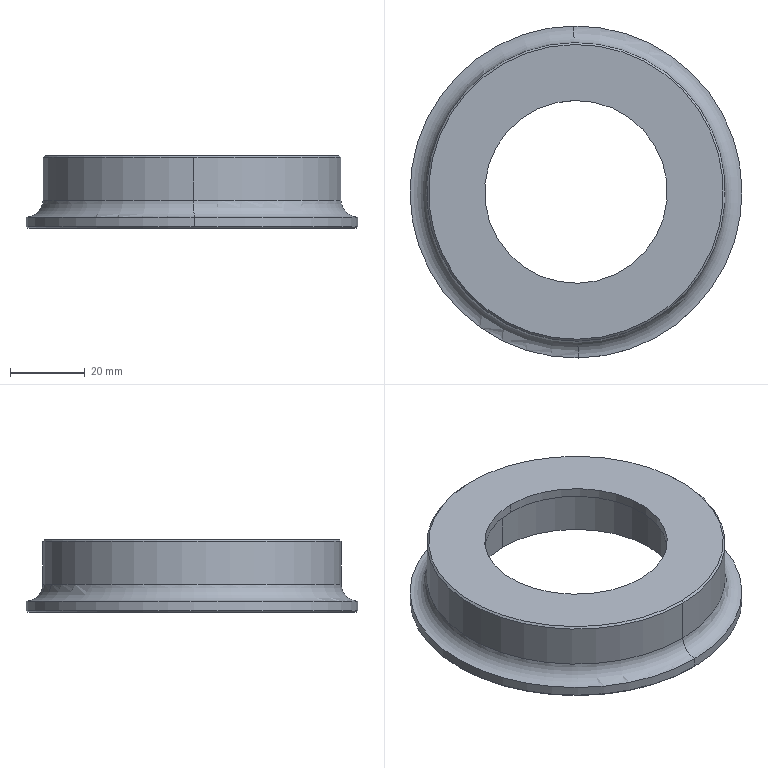Component | SolidWorks | 12AInnerSideWheel-EngravingAndMillingAxis-2_12AInnerSideWheel-2 | 1 solid | 20 faces | box 89 x 89 x 19.5 mm | volume 50313 mm3 | cylinder 10 | cone 4 | plane 4 | torus 2 | commonest cylinder face diameters 89 x2 73 x2 55 x2 49 x2 80 x2 | material Cr12MoV
build123d program:
from build123d import *

# Parameters (mm, degrees)
CHAMFER1_SIZE = 0.5
CHAMFER2_SIZE = 0.5


with BuildPart() as part:
    # Sketch1 → Revolve1 (revolve)
    with BuildSketch(Plane.XY, mode=Mode.PRIVATE) as revolve1_sk:
        with BuildLine():
            Line((27.5, 15.5), (27.5, 2.5))
            Line((27.5, 2.5), (24.5, 2.5))
            Line((24.5, 2.5), (24.5, 0))
            Line((24.5, 0), (40, 0))
            Line((40, 0), (40, 12))
            ThreePointArc((40, 12), (41.318, 15.182), (44.5, 16.5))
            Line((44.5, 16.5), (44.5, 19.5))
            Line((44.5, 19.5), (36.5, 19.5))
            Line((36.5, 19.5), (36.5, 15.5))
            Line((36.5, 15.5), (27.5, 15.5))
        make_face()
    revolve(revolve1_sk.sketch.rotate(Axis((0, 0, 0), (0, 1, 0)), 90), axis=Axis((0, 0, 0), (0, 1, 0)))

    # Chamfer1
    chamfer1_edges = [part.edges().sort_by_distance(p)[0] for p in [
        (0, 19.5, 44.5),
    ]]
    chamfer(chamfer1_edges, length=CHAMFER1_SIZE)

    # Chamfer2
    chamfer2_edges = [part.edges().sort_by_distance(p)[0] for p in [
        (0, 0, 40),
    ]]
    chamfer(chamfer2_edges, length=CHAMFER2_SIZE)


solid = part.part

# Placed as in the assembly
solid = solid.moved(Location((406.598, 137.038, 36.75), (-90, 0, 0)))
STEP:
#1=COLOUR_RGB('',0.7922,0.8196,0.9333);
#2=FILL_AREA_STYLE_COLOUR('',#1);
#3=FILL_AREA_STYLE('',(#2));
#4=SURFACE_STYLE_FILL_AREA(#3);
#5=SURFACE_SIDE_STYLE('',(#4));
#6=SURFACE_STYLE_USAGE(.BOTH.,#5);
#7=PRESENTATION_STYLE_ASSIGNMENT((#6));
#8=CARTESIAN_POINT('',(16.028,3.84,1.447));
#9=VERTEX_POINT('',#8);
#10=CARTESIAN_POINT('',(15.988,6.95,1.447));
#11=VERTEX_POINT('',#10);
#12=CARTESIAN_POINT('',(16.008,5.395,1.447));
#13=DIRECTION('',(-0.,-0.,1.));
#14=DIRECTION('',(0.01289,-0.9999,0.));
#15=AXIS2_PLACEMENT_3D('',#12,#13,#14);
#16=CIRCLE('',#15,1.555);
#17=EDGE_CURVE('',#9,#11,#16,.T.);
#18=ORIENTED_EDGE('',*,*,#17,.F.);
#19=CARTESIAN_POINT('',(16.028,3.821,1.427));
#20=VERTEX_POINT('',#19);
#21=CARTESIAN_POINT('',(16.028,3.84,1.447));
#22=DIRECTION('',(0.009113,-0.707,-0.7071));
#23=VECTOR('',#22,39.37);
#24=LINE('',#21,#23);
#25=EDGE_CURVE('',#9,#20,#24,.T.);
#26=ORIENTED_EDGE('',*,*,#25,.T.);
#27=CARTESIAN_POINT('',(15.988,6.97,1.427));
#28=VERTEX_POINT('',#27);
#29=CARTESIAN_POINT('',(16.008,5.395,1.427));
#30=DIRECTION('',(0.,0.,-1.));
#31=DIRECTION('',(0.01289,-0.9999,0.));
#32=AXIS2_PLACEMENT_3D('',#29,#30,#31);
#33=CIRCLE('',#32,1.575);
#34=EDGE_CURVE('',#28,#20,#33,.T.);
#35=ORIENTED_EDGE('',*,*,#34,.F.);
#36=CARTESIAN_POINT('',(15.988,6.95,1.447));
#37=DIRECTION('',(-0.009113,0.707,-0.7071));
#38=VECTOR('',#37,39.37);
#39=LINE('',#36,#38);
#40=EDGE_CURVE('',#11,#28,#39,.T.);
#41=ORIENTED_EDGE('',*,*,#40,.F.);
#42=EDGE_LOOP('',(#18,#26,#35,#41));
#43=FACE_OUTER_BOUND('',#42,.T.);
#44=CARTESIAN_POINT('',(16.008,5.395,1.447));
#45=DIRECTION('',(0.,0.,-1.));
#46=DIRECTION('',(-0.01289,0.9999,0.));
#47=AXIS2_PLACEMENT_3D('',#44,#45,#46);
#48=CONICAL_SURFACE('',#47,1.555,0.7854);
#49=ADVANCED_FACE('',(#43),#48,.T.);
#50=CARTESIAN_POINT('',(15.985,7.127,0.6791));
#51=VERTEX_POINT('',#50);
#52=CARTESIAN_POINT('',(16.03,3.663,0.6791));
#53=VERTEX_POINT('',#52);
#54=CARTESIAN_POINT('',(16.008,5.395,0.6791));
#55=DIRECTION('',(0.,0.,-1.));
#56=DIRECTION('',(-0.01289,0.9999,0.));
#57=AXIS2_PLACEMENT_3D('',#54,#55,#56);
#58=CIRCLE('',#57,1.732);
#59=EDGE_CURVE('',#51,#53,#58,.T.);
#60=ORIENTED_EDGE('',*,*,#59,.F.);
#61=CARTESIAN_POINT('',(15.985,7.147,0.6988));
#62=VERTEX_POINT('',#61);
#63=CARTESIAN_POINT('',(15.985,7.147,0.6988));
#64=DIRECTION('',(-0.009113,0.707,0.7071));
#65=VECTOR('',#64,39.37);
#66=LINE('',#63,#65);
#67=EDGE_CURVE('',#51,#62,#66,.T.);
#68=ORIENTED_EDGE('',*,*,#67,.T.);
#69=CARTESIAN_POINT('',(16.03,3.643,0.6988));
#70=VERTEX_POINT('',#69);
#71=CARTESIAN_POINT('',(16.008,5.395,0.6988));
#72=DIRECTION('',(-0.,-0.,1.));
#73=DIRECTION('',(-0.01289,0.9999,0.));
#74=AXIS2_PLACEMENT_3D('',#71,#72,#73);
#75=CIRCLE('',#74,1.752);
#76=EDGE_CURVE('',#70,#62,#75,.T.);
#77=ORIENTED_EDGE('',*,*,#76,.F.);
#78=CARTESIAN_POINT('',(16.03,3.643,0.6988));
#79=DIRECTION('',(0.009113,-0.707,0.7071));
#80=VECTOR('',#79,39.37);
#81=LINE('',#78,#80);
#82=EDGE_CURVE('',#53,#70,#81,.T.);
#83=ORIENTED_EDGE('',*,*,#82,.F.);
#84=EDGE_LOOP('',(#60,#68,#77,#83));
#85=FACE_OUTER_BOUND('',#84,.T.);
#86=CARTESIAN_POINT('',(16.008,5.395,0.6988));
#87=DIRECTION('',(-0.,-0.,1.));
#88=DIRECTION('',(0.01289,-0.9999,0.));
#89=AXIS2_PLACEMENT_3D('',#86,#87,#88);
#90=CONICAL_SURFACE('',#89,1.752,0.7854);
#91=ADVANCED_FACE('',(#85),#90,.T.);
#92=ORIENTED_EDGE('',*,*,#76,.T.);
#93=CARTESIAN_POINT('',(15.985,7.147,0.7972));
#94=VERTEX_POINT('',#93);
#95=CARTESIAN_POINT('',(15.985,7.147,1.447));
#96=DIRECTION('',(-0.,-0.,1.));
#97=VECTOR('',#96,39.37);
#98=LINE('',#95,#97);
#99=EDGE_CURVE('',#62,#94,#98,.T.);
#100=ORIENTED_EDGE('',*,*,#99,.T.);
#101=CARTESIAN_POINT('',(16.03,3.643,0.7972));
#102=VERTEX_POINT('',#101);
#103=CARTESIAN_POINT('',(16.008,5.395,0.7972));
#104=DIRECTION('',(-0.,-0.,1.));
#105=DIRECTION('',(0.01289,-0.9999,0.));
#106=AXIS2_PLACEMENT_3D('',#103,#104,#105);
#107=CIRCLE('',#106,1.752);
#108=EDGE_CURVE('',#102,#94,#107,.T.);
#109=ORIENTED_EDGE('',*,*,#108,.F.);
#110=CARTESIAN_POINT('',(16.03,3.643,1.447));
#111=DIRECTION('',(-0.,-0.,1.));
#112=VECTOR('',#111,39.37);
#113=LINE('',#110,#112);
#114=EDGE_CURVE('',#70,#102,#113,.T.);
#115=ORIENTED_EDGE('',*,*,#114,.F.);
#116=EDGE_LOOP('',(#92,#100,#109,#115));
#117=FACE_OUTER_BOUND('',#116,.T.);
#118=CARTESIAN_POINT('',(16.008,5.395,1.447));
#119=DIRECTION('',(-0.,-0.,1.));
#120=DIRECTION('',(0.01289,-0.9999,0.));
#121=AXIS2_PLACEMENT_3D('',#118,#119,#120);
#122=CYLINDRICAL_SURFACE('',#121,1.752);
#123=ADVANCED_FACE('',(#117),#122,.T.);
#124=CARTESIAN_POINT('',(15.989,6.832,0.6791));
#125=VERTEX_POINT('',#124);
#126=CARTESIAN_POINT('',(16.026,3.958,0.6791));
#127=VERTEX_POINT('',#126);
#128=CARTESIAN_POINT('',(16.008,5.395,0.6791));
#129=DIRECTION('',(-0.,-0.,1.));
#130=DIRECTION('',(0.01289,-0.9999,0.));
#131=AXIS2_PLACEMENT_3D('',#128,#129,#130);
#132=CIRCLE('',#131,1.437);
#133=EDGE_CURVE('',#125,#127,#132,.T.);
#134=ORIENTED_EDGE('',*,*,#133,.F.);
#135=CARTESIAN_POINT('',(15.989,6.832,0.8366));
#136=VERTEX_POINT('',#135);
#137=CARTESIAN_POINT('',(15.989,6.832,1.447));
#138=DIRECTION('',(-0.,-0.,1.));
#139=VECTOR('',#138,39.37);
#140=LINE('',#137,#139);
#141=EDGE_CURVE('',#125,#136,#140,.T.);
#142=ORIENTED_EDGE('',*,*,#141,.T.);
#143=CARTESIAN_POINT('',(16.026,3.958,0.8366));
#144=VERTEX_POINT('',#143);
#145=CARTESIAN_POINT('',(16.008,5.395,0.8366));
#146=DIRECTION('',(-0.,-0.,1.));
#147=DIRECTION('',(0.01289,-0.9999,0.));
#148=AXIS2_PLACEMENT_3D('',#145,#146,#147);
#149=CIRCLE('',#148,1.437);
#150=EDGE_CURVE('',#136,#144,#149,.T.);
#151=ORIENTED_EDGE('',*,*,#150,.T.);
#152=CARTESIAN_POINT('',(16.026,3.958,1.447));
#153=DIRECTION('',(-0.,-0.,1.));
#154=VECTOR('',#153,39.37);
#155=LINE('',#152,#154);
#156=EDGE_CURVE('',#127,#144,#155,.T.);
#157=ORIENTED_EDGE('',*,*,#156,.F.);
#158=EDGE_LOOP('',(#134,#142,#151,#157));
#159=FACE_OUTER_BOUND('',#158,.T.);
#160=CARTESIAN_POINT('',(16.008,5.395,1.447));
#161=DIRECTION('',(-0.,-0.,1.));
#162=DIRECTION('',(0.01289,-0.9999,0.));
#163=AXIS2_PLACEMENT_3D('',#160,#161,#162);
#164=CYLINDRICAL_SURFACE('',#163,1.437);
#165=ADVANCED_FACE('',(#159),#164,.F.);
#166=CARTESIAN_POINT('',(15.994,6.478,0.8366));
#167=VERTEX_POINT('',#166);
#168=CARTESIAN_POINT('',(16.022,4.313,0.8366));
#169=VERTEX_POINT('',#168);
#170=CARTESIAN_POINT('',(16.008,5.395,0.8366));
#171=DIRECTION('',(-0.,-0.,1.));
#172=DIRECTION('',(0.01289,-0.9999,0.));
#173=AXIS2_PLACEMENT_3D('',#170,#171,#172);
#174=CIRCLE('',#173,1.083);
#175=EDGE_CURVE('',#167,#169,#174,.T.);
#176=ORIENTED_EDGE('',*,*,#175,.F.);
#177=CARTESIAN_POINT('',(15.994,6.478,1.348));
#178=VERTEX_POINT('',#177);
#179=CARTESIAN_POINT('',(15.994,6.478,1.447));
#180=DIRECTION('',(-0.,-0.,1.));
#181=VECTOR('',#180,39.37);
#182=LINE('',#179,#181);
#183=EDGE_CURVE('',#167,#178,#182,.T.);
#184=ORIENTED_EDGE('',*,*,#183,.T.);
#185=CARTESIAN_POINT('',(16.022,4.313,1.348));
#186=VERTEX_POINT('',#185);
#187=CARTESIAN_POINT('',(16.008,5.395,1.348));
#188=DIRECTION('',(-0.,-0.,1.));
#189=DIRECTION('',(0.01289,-0.9999,0.));
#190=AXIS2_PLACEMENT_3D('',#187,#188,#189);
#191=CIRCLE('',#190,1.083);
#192=EDGE_CURVE('',#178,#186,#191,.T.);
#193=ORIENTED_EDGE('',*,*,#192,.T.);
#194=CARTESIAN_POINT('',(16.022,4.313,1.447));
#195=DIRECTION('',(-0.,-0.,1.));
#196=VECTOR('',#195,39.37);
#197=LINE('',#194,#196);
#198=EDGE_CURVE('',#169,#186,#197,.T.);
#199=ORIENTED_EDGE('',*,*,#198,.F.);
#200=EDGE_LOOP('',(#176,#184,#193,#199));
#201=FACE_OUTER_BOUND('',#200,.T.);
#202=CARTESIAN_POINT('',(16.008,5.395,1.447));
#203=DIRECTION('',(-0.,-0.,1.));
#204=DIRECTION('',(0.01289,-0.9999,0.));
#205=AXIS2_PLACEMENT_3D('',#202,#203,#204);
#206=CYLINDRICAL_SURFACE('',#205,1.083);
#207=ADVANCED_FACE('',(#201),#206,.F.);
#208=CARTESIAN_POINT('',(15.995,6.36,1.348));
#209=VERTEX_POINT('',#208);
#210=CARTESIAN_POINT('',(16.02,4.431,1.348));
#211=VERTEX_POINT('',#210);
#212=CARTESIAN_POINT('',(16.008,5.395,1.348));
#213=DIRECTION('',(-0.,-0.,1.));
#214=DIRECTION('',(0.01289,-0.9999,0.));
#215=AXIS2_PLACEMENT_3D('',#212,#213,#214);
#216=CIRCLE('',#215,0.9646);
#217=EDGE_CURVE('',#209,#211,#216,.T.);
#218=ORIENTED_EDGE('',*,*,#217,.F.);
#219=CARTESIAN_POINT('',(15.995,6.36,1.447));
#220=VERTEX_POINT('',#219);
#221=CARTESIAN_POINT('',(15.995,6.36,1.447));
#222=DIRECTION('',(-0.,-0.,1.));
#223=VECTOR('',#222,39.37);
#224=LINE('',#221,#223);
#225=EDGE_CURVE('',#209,#220,#224,.T.);
#226=ORIENTED_EDGE('',*,*,#225,.T.);
#227=CARTESIAN_POINT('',(16.02,4.431,1.447));
#228=VERTEX_POINT('',#227);
#229=CARTESIAN_POINT('',(16.008,5.395,1.447));
#230=DIRECTION('',(-0.,-0.,1.));
#231=DIRECTION('',(0.01289,-0.9999,0.));
#232=AXIS2_PLACEMENT_3D('',#229,#230,#231);
#233=CIRCLE('',#232,0.9646);
#234=EDGE_CURVE('',#220,#228,#233,.T.);
#235=ORIENTED_EDGE('',*,*,#234,.T.);
#236=CARTESIAN_POINT('',(16.02,4.431,1.447));
#237=DIRECTION('',(-0.,-0.,1.));
#238=VECTOR('',#237,39.37);
#239=LINE('',#236,#238);
#240=EDGE_CURVE('',#211,#228,#239,.T.);
#241=ORIENTED_EDGE('',*,*,#240,.F.);
#242=EDGE_LOOP('',(#218,#226,#235,#241));
#243=FACE_OUTER_BOUND('',#242,.T.);
#244=CARTESIAN_POINT('',(16.008,5.395,1.447));
#245=DIRECTION('',(-0.,-0.,1.));
#246=DIRECTION('',(0.01289,-0.9999,0.));
#247=AXIS2_PLACEMENT_3D('',#244,#245,#246);
#248=CYLINDRICAL_SURFACE('',#247,0.9646);
#249=ADVANCED_FACE('',(#243),#248,.F.);
#250=CARTESIAN_POINT('',(16.028,3.821,0.9744));
#251=VERTEX_POINT('',#250);
#252=CARTESIAN_POINT('',(15.988,6.97,0.9744));
#253=VERTEX_POINT('',#252);
#254=CARTESIAN_POINT('',(16.008,5.395,0.9744));
#255=DIRECTION('',(-0.,-0.,1.));
#256=DIRECTION('',(0.01289,-0.9999,0.));
#257=AXIS2_PLACEMENT_3D('',#254,#255,#256);
#258=CIRCLE('',#257,1.575);
#259=EDGE_CURVE('',#251,#253,#258,.T.);
#260=ORIENTED_EDGE('',*,*,#259,.T.);
#261=CARTESIAN_POINT('',(15.988,6.97,1.447));
#262=DIRECTION('',(-0.,-0.,1.));
#263=VECTOR('',#262,39.37);
#264=LINE('',#261,#263);
#265=EDGE_CURVE('',#253,#28,#264,.T.);
#266=ORIENTED_EDGE('',*,*,#265,.T.);
#267=ORIENTED_EDGE('',*,*,#34,.T.);
#268=CARTESIAN_POINT('',(16.028,3.821,1.447));
#269=DIRECTION('',(-0.,-0.,1.));
#270=VECTOR('',#269,39.37);
#271=LINE('',#268,#270);
#272=EDGE_CURVE('',#251,#20,#271,.T.);
#273=ORIENTED_EDGE('',*,*,#272,.F.);
#274=EDGE_LOOP('',(#260,#266,#267,#273));
#275=FACE_OUTER_BOUND('',#274,.T.);
#276=CARTESIAN_POINT('',(16.008,5.395,1.447));
#277=DIRECTION('',(-0.,-0.,1.));
#278=DIRECTION('',(0.01289,-0.9999,0.));
#279=AXIS2_PLACEMENT_3D('',#276,#277,#278);
#280=CYLINDRICAL_SURFACE('',#279,1.575);
#281=ADVANCED_FACE('',(#275),#280,.T.);
#282=CARTESIAN_POINT('',(16.008,5.395,0.9744));
#283=DIRECTION('',(-0.,-0.,1.));
#284=DIRECTION('',(0.01289,-0.9999,0.));
#285=AXIS2_PLACEMENT_3D('',#282,#283,#284);
#286=CIRCLE('',#285,1.575);
#287=EDGE_CURVE('',#253,#251,#286,.T.);
#288=ORIENTED_EDGE('',*,*,#287,.F.);
#289=CARTESIAN_POINT('',(15.985,7.147,0.9744));
#290=DIRECTION('',(0.9999,0.01289,0.));
#291=DIRECTION('',(-0.01289,0.9999,0.));
#292=AXIS2_PLACEMENT_3D('',#289,#290,#291);
#293=CIRCLE('',#292,0.1772);
#294=EDGE_CURVE('',#253,#94,#293,.T.);
#295=ORIENTED_EDGE('',*,*,#294,.T.);
#296=CARTESIAN_POINT('',(16.008,5.395,0.7972));
#297=DIRECTION('',(-0.,-0.,1.));
#298=DIRECTION('',(0.01289,-0.9999,0.));
#299=AXIS2_PLACEMENT_3D('',#296,#297,#298);
#300=CIRCLE('',#299,1.752);
#301=EDGE_CURVE('',#94,#102,#300,.T.);
#302=ORIENTED_EDGE('',*,*,#301,.T.);
#303=CARTESIAN_POINT('',(16.03,3.643,0.9744));
#304=DIRECTION('',(-0.9999,-0.01289,-0.));
#305=DIRECTION('',(0.01289,-0.9999,0.));
#306=AXIS2_PLACEMENT_3D('',#303,#304,#305);
#307=CIRCLE('',#306,0.1772);
#308=EDGE_CURVE('',#251,#102,#307,.T.);
#309=ORIENTED_EDGE('',*,*,#308,.F.);
#310=EDGE_LOOP('',(#288,#295,#302,#309));
#311=FACE_OUTER_BOUND('',#310,.T.);
#312=CARTESIAN_POINT('',(16.008,5.395,0.9744));
#313=DIRECTION('',(-0.,-0.,1.));
#314=DIRECTION('',(0.01289,-0.9999,-0.));
#315=AXIS2_PLACEMENT_3D('',#312,#313,#314);
#316=TOROIDAL_SURFACE('',#315,1.752,0.1772);
#317=ADVANCED_FACE('',(#311),#316,.F.);
#318=ORIENTED_EDGE('',*,*,#294,.F.);
#319=ORIENTED_EDGE('',*,*,#259,.F.);
#320=ORIENTED_EDGE('',*,*,#308,.T.);
#321=ORIENTED_EDGE('',*,*,#108,.T.);
#322=EDGE_LOOP('',(#318,#319,#320,#321));
#323=FACE_OUTER_BOUND('',#322,.T.);
#324=CARTESIAN_POINT('',(16.008,5.395,0.9744));
#325=DIRECTION('',(-0.,-0.,1.));
#326=DIRECTION('',(0.01289,-0.9999,-0.));
#327=AXIS2_PLACEMENT_3D('',#324,#325,#326);
#328=TOROIDAL_SURFACE('',#327,1.752,0.1772);
#329=ADVANCED_FACE('',(#323),#328,.F.);
#330=ORIENTED_EDGE('',*,*,#265,.F.);
#331=ORIENTED_EDGE('',*,*,#287,.T.);
#332=ORIENTED_EDGE('',*,*,#272,.T.);
#333=CARTESIAN_POINT('',(16.008,5.395,1.427));
#334=DIRECTION('',(0.,0.,-1.));
#335=DIRECTION('',(0.01289,-0.9999,0.));
#336=AXIS2_PLACEMENT_3D('',#333,#334,#335);
#337=CIRCLE('',#336,1.575);
#338=EDGE_CURVE('',#20,#28,#337,.T.);
#339=ORIENTED_EDGE('',*,*,#338,.T.);
#340=EDGE_LOOP('',(#330,#331,#332,#339));
#341=FACE_OUTER_BOUND('',#340,.T.);
#342=CARTESIAN_POINT('',(16.008,5.395,1.447));
#343=DIRECTION('',(-0.,-0.,1.));
#344=DIRECTION('',(0.01289,-0.9999,0.));
#345=AXIS2_PLACEMENT_3D('',#342,#343,#344);
#346=CYLINDRICAL_SURFACE('',#345,1.575);
#347=ADVANCED_FACE('',(#341),#346,.T.);
#348=CARTESIAN_POINT('',(16.008,5.395,1.447));
#349=DIRECTION('',(-0.,-0.,1.));
#350=DIRECTION('',(0.01289,-0.9999,0.));
#351=AXIS2_PLACEMENT_3D('',#348,#349,#350);
#352=CIRCLE('',#351,1.555);
#353=EDGE_CURVE('',#11,#9,#352,.T.);
#354=ORIENTED_EDGE('',*,*,#353,.T.);
#355=ORIENTED_EDGE('',*,*,#17,.T.);
#356=EDGE_LOOP('',(#354,#355));
#357=FACE_OUTER_BOUND('',#356,.T.);
#358=CARTESIAN_POINT('',(16.008,5.395,1.447));
#359=DIRECTION('',(-0.,-0.,1.));
#360=DIRECTION('',(0.01289,-0.9999,0.));
#361=AXIS2_PLACEMENT_3D('',#358,#359,#360);
#362=CIRCLE('',#361,0.9646);
#363=EDGE_CURVE('',#228,#220,#362,.T.);
#364=ORIENTED_EDGE('',*,*,#363,.F.);
#365=ORIENTED_EDGE('',*,*,#234,.F.);
#366=EDGE_LOOP('',(#364,#365));
#367=FACE_BOUND('',#366,.T.);
#368=CARTESIAN_POINT('',(16.972,5.408,1.447));
#369=DIRECTION('',(-0.,-0.,1.));
#370=DIRECTION('',(0.01289,-0.9999,-0.));
#371=AXIS2_PLACEMENT_3D('',#368,#369,#370);
#372=PLANE('',#371);
#373=ADVANCED_FACE('',(#357,#367),#372,.T.);
#374=ORIENTED_EDGE('',*,*,#225,.F.);
#375=CARTESIAN_POINT('',(16.008,5.395,1.348));
#376=DIRECTION('',(-0.,-0.,1.));
#377=DIRECTION('',(0.01289,-0.9999,0.));
#378=AXIS2_PLACEMENT_3D('',#375,#376,#377);
#379=CIRCLE('',#378,0.9646);
#380=EDGE_CURVE('',#211,#209,#379,.T.);
#381=ORIENTED_EDGE('',*,*,#380,.F.);
#382=ORIENTED_EDGE('',*,*,#240,.T.);
#383=ORIENTED_EDGE('',*,*,#363,.T.);
#384=EDGE_LOOP('',(#374,#381,#382,#383));
#385=FACE_OUTER_BOUND('',#384,.T.);
#386=CARTESIAN_POINT('',(16.008,5.395,1.447));
#387=DIRECTION('',(-0.,-0.,1.));
#388=DIRECTION('',(0.01289,-0.9999,0.));
#389=AXIS2_PLACEMENT_3D('',#386,#387,#388);
#390=CYLINDRICAL_SURFACE('',#389,0.9646);
#391=ADVANCED_FACE('',(#385),#390,.F.);
#392=ORIENTED_EDGE('',*,*,#380,.T.);
#393=ORIENTED_EDGE('',*,*,#217,.T.);
#394=EDGE_LOOP('',(#392,#393));
#395=FACE_BOUND('',#394,.T.);
#396=CARTESIAN_POINT('',(16.008,5.395,1.348));
#397=DIRECTION('',(-0.,-0.,1.));
#398=DIRECTION('',(0.01289,-0.9999,0.));
#399=AXIS2_PLACEMENT_3D('',#396,#397,#398);
#400=CIRCLE('',#399,1.083);
#401=EDGE_CURVE('',#186,#178,#400,.T.);
#402=ORIENTED_EDGE('',*,*,#401,.F.);
#403=ORIENTED_EDGE('',*,*,#192,.F.);
#404=EDGE_LOOP('',(#402,#403));
#405=FACE_OUTER_BOUND('',#404,.T.);
#406=CARTESIAN_POINT('',(17.09,5.409,1.348));
#407=DIRECTION('',(0.,0.,-1.));
#408=DIRECTION('',(-0.01289,0.9999,0.));
#409=AXIS2_PLACEMENT_3D('',#406,#407,#408);
#410=PLANE('',#409);
#411=ADVANCED_FACE('',(#395,#405),#410,.T.);
#412=ORIENTED_EDGE('',*,*,#183,.F.);
#413=CARTESIAN_POINT('',(16.008,5.395,0.8366));
#414=DIRECTION('',(-0.,-0.,1.));
#415=DIRECTION('',(0.01289,-0.9999,0.));
#416=AXIS2_PLACEMENT_3D('',#413,#414,#415);
#417=CIRCLE('',#416,1.083);
#418=EDGE_CURVE('',#169,#167,#417,.T.);
#419=ORIENTED_EDGE('',*,*,#418,.F.);
#420=ORIENTED_EDGE('',*,*,#198,.T.);
#421=ORIENTED_EDGE('',*,*,#401,.T.);
#422=EDGE_LOOP('',(#412,#419,#420,#421));
#423=FACE_OUTER_BOUND('',#422,.T.);
#424=CARTESIAN_POINT('',(16.008,5.395,1.447));
#425=DIRECTION('',(-0.,-0.,1.));
#426=DIRECTION('',(0.01289,-0.9999,0.));
#427=AXIS2_PLACEMENT_3D('',#424,#425,#426);
#428=CYLINDRICAL_SURFACE('',#427,1.083);
#429=ADVANCED_FACE('',(#423),#428,.F.);
#430=ORIENTED_EDGE('',*,*,#418,.T.);
#431=ORIENTED_EDGE('',*,*,#175,.T.);
#432=EDGE_LOOP('',(#430,#431));
#433=FACE_BOUND('',#432,.T.);
#434=CARTESIAN_POINT('',(16.008,5.395,0.8366));
#435=DIRECTION('',(-0.,-0.,1.));
#436=DIRECTION('',(0.01289,-0.9999,0.));
#437=AXIS2_PLACEMENT_3D('',#434,#435,#436);
#438=CIRCLE('',#437,1.437);
#439=EDGE_CURVE('',#144,#136,#438,.T.);
#440=ORIENTED_EDGE('',*,*,#439,.F.);
#441=ORIENTED_EDGE('',*,*,#150,.F.);
#442=EDGE_LOOP('',(#440,#441));
#443=FACE_OUTER_BOUND('',#442,.T.);
#444=CARTESIAN_POINT('',(17.445,5.414,0.8366));
#445=DIRECTION('',(0.,0.,-1.));
#446=DIRECTION('',(-0.01289,0.9999,0.));
#447=AXIS2_PLACEMENT_3D('',#444,#445,#446);
#448=PLANE('',#447);
#449=ADVANCED_FACE('',(#433,#443),#448,.T.);
#450=ORIENTED_EDGE('',*,*,#141,.F.);
#451=CARTESIAN_POINT('',(16.008,5.395,0.6791));
#452=DIRECTION('',(-0.,-0.,1.));
#453=DIRECTION('',(0.01289,-0.9999,0.));
#454=AXIS2_PLACEMENT_3D('',#451,#452,#453);
#455=CIRCLE('',#454,1.437);
#456=EDGE_CURVE('',#127,#125,#455,.T.);
#457=ORIENTED_EDGE('',*,*,#456,.F.);
#458=ORIENTED_EDGE('',*,*,#156,.T.);
#459=ORIENTED_EDGE('',*,*,#439,.T.);
#460=EDGE_LOOP('',(#450,#457,#458,#459));
#461=FACE_OUTER_BOUND('',#460,.T.);
#462=CARTESIAN_POINT('',(16.008,5.395,1.447));
#463=DIRECTION('',(-0.,-0.,1.));
#464=DIRECTION('',(0.01289,-0.9999,0.));
#465=AXIS2_PLACEMENT_3D('',#462,#463,#464);
#466=CYLINDRICAL_SURFACE('',#465,1.437);
#467=ADVANCED_FACE('',(#461),#466,.F.);
#468=CARTESIAN_POINT('',(16.008,5.395,0.6791));
#469=DIRECTION('',(0.,0.,-1.));
#470=DIRECTION('',(-0.01289,0.9999,0.));
#471=AXIS2_PLACEMENT_3D('',#468,#469,#470);
#472=CIRCLE('',#471,1.732);
#473=EDGE_CURVE('',#53,#51,#472,.T.);
#474=ORIENTED_EDGE('',*,*,#473,.T.);
#475=ORIENTED_EDGE('',*,*,#59,.T.);
#476=EDGE_LOOP('',(#474,#475));
#477=FACE_OUTER_BOUND('',#476,.T.);
#478=ORIENTED_EDGE('',*,*,#456,.T.);
#479=ORIENTED_EDGE('',*,*,#133,.T.);
#480=EDGE_LOOP('',(#478,#479));
#481=FACE_BOUND('',#480,.T.);
#482=CARTESIAN_POINT('',(17.76,5.418,0.6791));
#483=DIRECTION('',(0.,0.,-1.));
#484=DIRECTION('',(-0.01289,0.9999,0.));
#485=AXIS2_PLACEMENT_3D('',#482,#483,#484);
#486=PLANE('',#485);
#487=ADVANCED_FACE('',(#477,#481),#486,.T.);
#488=ORIENTED_EDGE('',*,*,#99,.F.);
#489=CARTESIAN_POINT('',(16.008,5.395,0.6988));
#490=DIRECTION('',(-0.,-0.,1.));
#491=DIRECTION('',(-0.01289,0.9999,0.));
#492=AXIS2_PLACEMENT_3D('',#489,#490,#491);
#493=CIRCLE('',#492,1.752);
#494=EDGE_CURVE('',#62,#70,#493,.T.);
#495=ORIENTED_EDGE('',*,*,#494,.T.);
#496=ORIENTED_EDGE('',*,*,#114,.T.);
#497=ORIENTED_EDGE('',*,*,#301,.F.);
#498=EDGE_LOOP('',(#488,#495,#496,#497));
#499=FACE_OUTER_BOUND('',#498,.T.);
#500=CARTESIAN_POINT('',(16.008,5.395,1.447));
#501=DIRECTION('',(-0.,-0.,1.));
#502=DIRECTION('',(0.01289,-0.9999,0.));
#503=AXIS2_PLACEMENT_3D('',#500,#501,#502);
#504=CYLINDRICAL_SURFACE('',#503,1.752);
#505=ADVANCED_FACE('',(#499),#504,.T.);
#506=ORIENTED_EDGE('',*,*,#67,.F.);
#507=ORIENTED_EDGE('',*,*,#473,.F.);
#508=ORIENTED_EDGE('',*,*,#82,.T.);
#509=ORIENTED_EDGE('',*,*,#494,.F.);
#510=EDGE_LOOP('',(#506,#507,#508,#509));
#511=FACE_OUTER_BOUND('',#510,.T.);
#512=CARTESIAN_POINT('',(16.008,5.395,0.6988));
#513=DIRECTION('',(-0.,-0.,1.));
#514=DIRECTION('',(0.01289,-0.9999,0.));
#515=AXIS2_PLACEMENT_3D('',#512,#513,#514);
#516=CONICAL_SURFACE('',#515,1.752,0.7854);
#517=ADVANCED_FACE('',(#511),#516,.T.);
#518=ORIENTED_EDGE('',*,*,#25,.F.);
#519=ORIENTED_EDGE('',*,*,#353,.F.);
#520=ORIENTED_EDGE('',*,*,#40,.T.);
#521=ORIENTED_EDGE('',*,*,#338,.F.);
#522=EDGE_LOOP('',(#518,#519,#520,#521));
#523=FACE_OUTER_BOUND('',#522,.T.);
#524=CARTESIAN_POINT('',(16.008,5.395,1.447));
#525=DIRECTION('',(0.,0.,-1.));
#526=DIRECTION('',(-0.01289,0.9999,0.));
#527=AXIS2_PLACEMENT_3D('',#524,#525,#526);
#528=CONICAL_SURFACE('',#527,1.555,0.7854);
#529=ADVANCED_FACE('',(#523),#528,.T.);
#530=CLOSED_SHELL('',(#49,#91,#123,#165,#207,#249,#281,#317,#329,#347,#373,#391,#411,#429,#449,#467,#487,#505,#517,#529));
#531=MANIFOLD_SOLID_BREP('',#530);
#532=STYLED_ITEM('',(#7),#531);
#533=PRESENTATION_LAYER_ASSIGNMENT('','',(#532));
#534=CARTESIAN_POINT('',(0.,0.,0.));
#535=DIRECTION('',(0.,0.,1.));
#536=DIRECTION('',(1.,0.,0.));
#537=AXIS2_PLACEMENT_3D('',#534,#535,#536);
#538=(LENGTH_UNIT()NAMED_UNIT(*)SI_UNIT($,.METRE.));
#539=LENGTH_MEASURE_WITH_UNIT(LENGTH_MEASURE(0.0254),#538);
#540=DIMENSIONAL_EXPONENTS(1.,0.,0.,0.,0.,0.,0.);
#541=(CONVERSION_BASED_UNIT('',#539)LENGTH_UNIT()NAMED_UNIT(#540));
#542=UNCERTAINTY_MEASURE_WITH_UNIT(LENGTH_MEASURE(0.00001),#541,'','');
#543=(NAMED_UNIT(*)PLANE_ANGLE_UNIT()SI_UNIT($,.RADIAN.));
#544=(NAMED_UNIT(*)SI_UNIT($,.STERADIAN.)SOLID_ANGLE_UNIT());
#545=(GEOMETRIC_REPRESENTATION_CONTEXT(3)GLOBAL_UNCERTAINTY_ASSIGNED_CONTEXT((#542))GLOBAL_UNIT_ASSIGNED_CONTEXT((#541,#543,#544))REPRESENTATION_CONTEXT('',''));
#546=ADVANCED_BREP_SHAPE_REPRESENTATION('',(#531,#537),#545);
#547=(LENGTH_UNIT()NAMED_UNIT(*)SI_UNIT($,.METRE.));
#548=LENGTH_MEASURE_WITH_UNIT(LENGTH_MEASURE(0.0254),#547);
#549=DIMENSIONAL_EXPONENTS(1.,0.,0.,0.,0.,0.,0.);
#550=(CONVERSION_BASED_UNIT('',#548)LENGTH_UNIT()NAMED_UNIT(#549));
#551=UNCERTAINTY_MEASURE_WITH_UNIT(LENGTH_MEASURE(0.00001),#550,'','');
#552=(NAMED_UNIT(*)PLANE_ANGLE_UNIT()SI_UNIT($,.RADIAN.));
#553=(NAMED_UNIT(*)SI_UNIT($,.STERADIAN.)SOLID_ANGLE_UNIT());
#554=(GEOMETRIC_REPRESENTATION_CONTEXT(3)GLOBAL_UNCERTAINTY_ASSIGNED_CONTEXT((#551))GLOBAL_UNIT_ASSIGNED_CONTEXT((#550,#552,#553))REPRESENTATION_CONTEXT('',''));
#555=MECHANICAL_DESIGN_GEOMETRIC_PRESENTATION_REPRESENTATION('',(#532),#554);